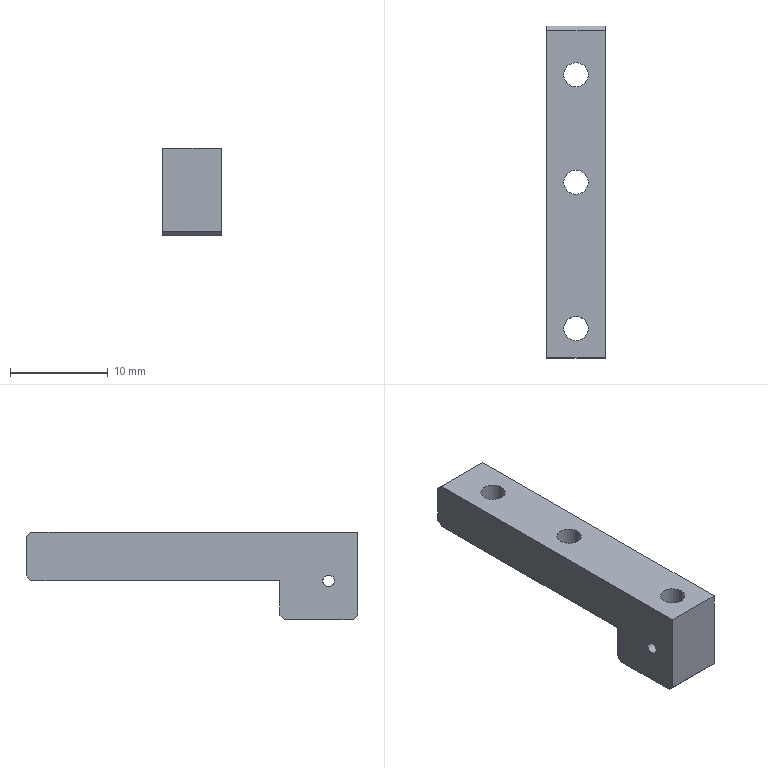Component | SolidWorks | 2018SOLIDWORKS1400000008-1 | 1 solid | 22 faces | box 6 x 34 x 9 mm | volume 1112 mm3 | plane 12 | cylinder 10 | commonest cylinder face diameters 2.5 x6 1.2 x4 | material Brass
build123d program:
from build123d import *

# Parameters (mm, degrees)
SKETCH1_W           = 12
SKETCH1_H           = 4
BOSS_EXTRUDE1_DEPTH = 3
SKETCH10_W          = 34
SKETCH10_H          = 6
BOSS_EXTRUDE2_DEPTH = 5
M3_TAPPED_HOLE1_D   = 2.5
SKETCH9_R           = 0.6
CUT_EXTRUDE7_DEPTH  = 30.479
CHAMFER1_SIZE       = 0.5
SKETCH14_W          = 4
SKETCH14_H          = 6
CUT_EXTRUDE8_DEPTH  = 4
CHAMFER2_SIZE       = 0.5
M3_TAPPED_HOLE2_D   = 2.5


with BuildPart() as part:
    # Sketch1 → Boss-Extrude1 (new, symmetric)
    with BuildSketch(Plane.XY):
        Rectangle(SKETCH1_W, SKETCH1_H)
    extrude(amount=BOSS_EXTRUDE1_DEPTH, both=True)

    # Sketch10 → Boss-Extrude2 (add)
    with BuildSketch(Plane(origin=(0, 2, 0), x_dir=(1, 0, 0), z_dir=(0, 1, 0))):
        with Locations((11, 0)):
            Rectangle(SKETCH10_W, SKETCH10_H)
    extrude(amount=BOSS_EXTRUDE2_DEPTH)

    # M3 Tapped Hole1 (through all)
    with Locations(Plane(origin=(0, 7, 0), x_dir=(1, 0, 0), z_dir=(0, 1, 0))):
        with Locations((12, 0), (23, 0)):
            Hole(M3_TAPPED_HOLE1_D / 2)

    # Sketch9 → Cut-Extrude7 (cut, through all)
    with BuildSketch(Plane.XY.offset(3)):
        with Locations((-3, 2)):
            Circle(SKETCH9_R)
    extrude(amount=-CUT_EXTRUDE7_DEPTH, mode=Mode.SUBTRACT)

    # Chamfer1
    chamfer1_edges = [part.edges().sort_by_distance(p)[0] for p in [
        (28, 7, 0),
        (28, 2, 0),
        (6, -2, 0),
        (-6, -2, 0),
    ]]
    chamfer(chamfer1_edges, length=CHAMFER1_SIZE)

    # Sketch14 → Cut-Extrude8 (cut)
    with BuildSketch(Plane.XZ.offset(2)):
        with Locations((4, 0)):
            Rectangle(SKETCH14_W, SKETCH14_H)
    extrude(amount=-CUT_EXTRUDE8_DEPTH, mode=Mode.SUBTRACT)

    # Chamfer2
    chamfer2_edges = [part.edges().sort_by_distance(p)[0] for p in [
        (2, -2, 0),
    ]]
    chamfer(chamfer2_edges, length=CHAMFER2_SIZE)

    # M3 Tapped Hole2 (through all)
    with Locations(Plane(origin=(0, 7, 0), x_dir=(1, 0, 0), z_dir=(0, 1, 0))):
        with Locations((-3, 0)):
            Hole(M3_TAPPED_HOLE2_D / 2)


solid = part.part

# Placed as in the assembly
solid = solid.moved(Location((84.712, -105.5, 215), (90, 90, 0)))
STEP:
#1=COLOUR_RGB('',0.7922,0.8196,0.9333);
#2=FILL_AREA_STYLE_COLOUR('',#1);
#3=FILL_AREA_STYLE('',(#2));
#4=SURFACE_STYLE_FILL_AREA(#3);
#5=SURFACE_SIDE_STYLE('',(#4));
#6=SURFACE_STYLE_USAGE(.BOTH.,#5);
#7=PRESENTATION_STYLE_ASSIGNMENT((#6));
#8=CARTESIAN_POINT('',(3.286,-4.272,8.386));
#9=VERTEX_POINT('',#8);
#10=CARTESIAN_POINT('',(3.384,-4.272,8.386));
#11=VERTEX_POINT('',#10);
#12=CARTESIAN_POINT('',(3.335,-4.272,8.386));
#13=DIRECTION('',(-0.,0.,1.));
#14=DIRECTION('',(1.,0.,0.));
#15=AXIS2_PLACEMENT_3D('',#12,#13,#14);
#16=CIRCLE('',#15,0.04921);
#17=EDGE_CURVE('',#9,#11,#16,.T.);
#18=ORIENTED_EDGE('',*,*,#17,.F.);
#19=CARTESIAN_POINT('',(3.286,-4.272,8.52));
#20=VERTEX_POINT('',#19);
#21=CARTESIAN_POINT('',(3.286,-4.272,8.74));
#22=DIRECTION('',(-0.,0.,1.));
#23=VECTOR('',#22,39.37);
#24=LINE('',#21,#23);
#25=EDGE_CURVE('',#9,#20,#24,.T.);
#26=ORIENTED_EDGE('',*,*,#25,.T.);
#27=CARTESIAN_POINT('',(3.292,-4.295,8.543));
#28=VERTEX_POINT('',#27);
#29=CARTESIAN_POINT('',(3.292,-4.295,8.543));
#30=CARTESIAN_POINT('',(3.292,-4.295,8.54));
#31=CARTESIAN_POINT('',(3.292,-4.295,8.537));
#32=CARTESIAN_POINT('',(3.29,-4.292,8.531));
#33=CARTESIAN_POINT('',(3.29,-4.291,8.529));
#34=CARTESIAN_POINT('',(3.288,-4.286,8.524));
#35=CARTESIAN_POINT('',(3.287,-4.284,8.523));
#36=CARTESIAN_POINT('',(3.286,-4.278,8.52));
#37=CARTESIAN_POINT('',(3.286,-4.275,8.52));
#38=CARTESIAN_POINT('',(3.286,-4.272,8.52));
#39=B_SPLINE_CURVE_WITH_KNOTS('',3,(#29,#30,#31,#32,#33,#34,#35,#36,#37,#38),.UNSPECIFIED.,.F.,.F.,(4,2,2,2,4),(0.001906,0.002143,0.002381,0.002619,0.002857),.UNSPECIFIED.);
#40=EDGE_CURVE('',#28,#20,#39,.T.);
#41=ORIENTED_EDGE('',*,*,#40,.F.);
#42=CARTESIAN_POINT('',(3.286,-4.272,8.567));
#43=VERTEX_POINT('',#42);
#44=CARTESIAN_POINT('',(3.286,-4.272,8.567));
#45=CARTESIAN_POINT('',(3.286,-4.275,8.567));
#46=CARTESIAN_POINT('',(3.286,-4.278,8.566));
#47=CARTESIAN_POINT('',(3.287,-4.284,8.564));
#48=CARTESIAN_POINT('',(3.288,-4.286,8.562));
#49=CARTESIAN_POINT('',(3.29,-4.291,8.558));
#50=CARTESIAN_POINT('',(3.29,-4.292,8.555));
#51=CARTESIAN_POINT('',(3.292,-4.295,8.55));
#52=CARTESIAN_POINT('',(3.292,-4.295,8.546));
#53=CARTESIAN_POINT('',(3.292,-4.295,8.543));
#54=B_SPLINE_CURVE_WITH_KNOTS('',3,(#44,#45,#46,#47,#48,#49,#50,#51,#52,#53),.UNSPECIFIED.,.F.,.F.,(4,2,2,2,4),(0.0009531,0.001191,0.001429,0.001667,0.001906),.UNSPECIFIED.);
#55=EDGE_CURVE('',#43,#28,#54,.T.);
#56=ORIENTED_EDGE('',*,*,#55,.F.);
#57=CARTESIAN_POINT('',(3.286,-4.272,8.74));
#58=VERTEX_POINT('',#57);
#59=CARTESIAN_POINT('',(3.286,-4.272,8.74));
#60=DIRECTION('',(-0.,0.,1.));
#61=VECTOR('',#60,39.37);
#62=LINE('',#59,#61);
#63=EDGE_CURVE('',#43,#58,#62,.T.);
#64=ORIENTED_EDGE('',*,*,#63,.T.);
#65=CARTESIAN_POINT('',(3.384,-4.272,8.74));
#66=VERTEX_POINT('',#65);
#67=CARTESIAN_POINT('',(3.335,-4.272,8.74));
#68=DIRECTION('',(-0.,0.,1.));
#69=DIRECTION('',(1.,0.,0.));
#70=AXIS2_PLACEMENT_3D('',#67,#68,#69);
#71=CIRCLE('',#70,0.04921);
#72=EDGE_CURVE('',#58,#66,#71,.T.);
#73=ORIENTED_EDGE('',*,*,#72,.T.);
#74=CARTESIAN_POINT('',(3.384,-4.272,8.567));
#75=VERTEX_POINT('',#74);
#76=CARTESIAN_POINT('',(3.384,-4.272,8.74));
#77=DIRECTION('',(-0.,0.,1.));
#78=VECTOR('',#77,39.37);
#79=LINE('',#76,#78);
#80=EDGE_CURVE('',#75,#66,#79,.T.);
#81=ORIENTED_EDGE('',*,*,#80,.F.);
#82=CARTESIAN_POINT('',(3.378,-4.295,8.543));
#83=VERTEX_POINT('',#82);
#84=CARTESIAN_POINT('',(3.378,-4.295,8.543));
#85=CARTESIAN_POINT('',(3.378,-4.295,8.546));
#86=CARTESIAN_POINT('',(3.379,-4.295,8.55));
#87=CARTESIAN_POINT('',(3.38,-4.292,8.555));
#88=CARTESIAN_POINT('',(3.381,-4.291,8.558));
#89=CARTESIAN_POINT('',(3.382,-4.286,8.562));
#90=CARTESIAN_POINT('',(3.383,-4.284,8.564));
#91=CARTESIAN_POINT('',(3.384,-4.278,8.566));
#92=CARTESIAN_POINT('',(3.384,-4.275,8.567));
#93=CARTESIAN_POINT('',(3.384,-4.272,8.567));
#94=B_SPLINE_CURVE_WITH_KNOTS('',3,(#84,#85,#86,#87,#88,#89,#90,#91,#92,#93),.UNSPECIFIED.,.F.,.F.,(4,2,2,2,4),(0.001906,0.002143,0.002381,0.002619,0.002857),.UNSPECIFIED.);
#95=EDGE_CURVE('',#83,#75,#94,.T.);
#96=ORIENTED_EDGE('',*,*,#95,.F.);
#97=CARTESIAN_POINT('',(3.384,-4.272,8.52));
#98=VERTEX_POINT('',#97);
#99=CARTESIAN_POINT('',(3.384,-4.272,8.52));
#100=CARTESIAN_POINT('',(3.384,-4.275,8.52));
#101=CARTESIAN_POINT('',(3.384,-4.278,8.52));
#102=CARTESIAN_POINT('',(3.383,-4.284,8.523));
#103=CARTESIAN_POINT('',(3.382,-4.286,8.524));
#104=CARTESIAN_POINT('',(3.381,-4.291,8.529));
#105=CARTESIAN_POINT('',(3.38,-4.292,8.531));
#106=CARTESIAN_POINT('',(3.379,-4.295,8.537));
#107=CARTESIAN_POINT('',(3.378,-4.295,8.54));
#108=CARTESIAN_POINT('',(3.378,-4.295,8.543));
#109=B_SPLINE_CURVE_WITH_KNOTS('',3,(#99,#100,#101,#102,#103,#104,#105,#106,#107,#108),.UNSPECIFIED.,.F.,.F.,(4,2,2,2,4),(0.0009531,0.001191,0.001429,0.001667,0.001906),.UNSPECIFIED.);
#110=EDGE_CURVE('',#98,#83,#109,.T.);
#111=ORIENTED_EDGE('',*,*,#110,.F.);
#112=CARTESIAN_POINT('',(3.384,-4.272,8.74));
#113=DIRECTION('',(-0.,0.,1.));
#114=VECTOR('',#113,39.37);
#115=LINE('',#112,#114);
#116=EDGE_CURVE('',#11,#98,#115,.T.);
#117=ORIENTED_EDGE('',*,*,#116,.F.);
#118=EDGE_LOOP('',(#18,#26,#41,#56,#64,#73,#81,#96,#111,#117));
#119=FACE_OUTER_BOUND('',#118,.T.);
#120=CARTESIAN_POINT('',(3.335,-4.272,8.74));
#121=DIRECTION('',(-0.,0.,1.));
#122=DIRECTION('',(1.,0.,0.));
#123=AXIS2_PLACEMENT_3D('',#120,#121,#122);
#124=CYLINDRICAL_SURFACE('',#123,0.04921);
#125=ADVANCED_FACE('',(#119),#124,.F.);
#126=CARTESIAN_POINT('',(3.378,-4.248,8.543));
#127=VERTEX_POINT('',#126);
#128=CARTESIAN_POINT('',(3.378,-4.248,8.543));
#129=CARTESIAN_POINT('',(3.378,-4.248,8.537));
#130=CARTESIAN_POINT('',(3.38,-4.251,8.531));
#131=CARTESIAN_POINT('',(3.382,-4.257,8.524));
#132=CARTESIAN_POINT('',(3.383,-4.26,8.523));
#133=CARTESIAN_POINT('',(3.384,-4.265,8.52));
#134=CARTESIAN_POINT('',(3.384,-4.269,8.52));
#135=CARTESIAN_POINT('',(3.384,-4.272,8.52));
#136=B_SPLINE_CURVE_WITH_KNOTS('',3,(#128,#129,#130,#131,#132,#133,#134,#135),.UNSPECIFIED.,.F.,.F.,(4,2,2,4),(0.,0.0004766,0.0007149,0.0009531),.UNSPECIFIED.);
#137=EDGE_CURVE('',#127,#98,#136,.T.);
#138=ORIENTED_EDGE('',*,*,#137,.T.);
#139=ORIENTED_EDGE('',*,*,#110,.T.);
#140=CARTESIAN_POINT('',(3.453,-4.295,8.543));
#141=VERTEX_POINT('',#140);
#142=CARTESIAN_POINT('',(3.217,-4.295,8.543));
#143=DIRECTION('',(1.,-0.,0.));
#144=VECTOR('',#143,39.37);
#145=LINE('',#142,#144);
#146=EDGE_CURVE('',#83,#141,#145,.T.);
#147=ORIENTED_EDGE('',*,*,#146,.T.);
#148=CARTESIAN_POINT('',(3.453,-4.248,8.543));
#149=VERTEX_POINT('',#148);
#150=CARTESIAN_POINT('',(3.453,-4.272,8.543));
#151=DIRECTION('',(1.,-0.,0.));
#152=DIRECTION('',(0.,1.,0.));
#153=AXIS2_PLACEMENT_3D('',#150,#151,#152);
#154=CIRCLE('',#153,0.02362);
#155=EDGE_CURVE('',#141,#149,#154,.T.);
#156=ORIENTED_EDGE('',*,*,#155,.T.);
#157=CARTESIAN_POINT('',(3.217,-4.248,8.543));
#158=DIRECTION('',(1.,-0.,0.));
#159=VECTOR('',#158,39.37);
#160=LINE('',#157,#159);
#161=EDGE_CURVE('',#127,#149,#160,.T.);
#162=ORIENTED_EDGE('',*,*,#161,.F.);
#163=EDGE_LOOP('',(#138,#139,#147,#156,#162));
#164=FACE_OUTER_BOUND('',#163,.T.);
#165=CARTESIAN_POINT('',(3.217,-4.272,8.543));
#166=DIRECTION('',(1.,-0.,0.));
#167=DIRECTION('',(0.,1.,0.));
#168=AXIS2_PLACEMENT_3D('',#165,#166,#167);
#169=CYLINDRICAL_SURFACE('',#168,0.02362);
#170=ADVANCED_FACE('',(#164),#169,.F.);
#171=CARTESIAN_POINT('',(3.286,-3.681,8.543));
#172=VERTEX_POINT('',#171);
#173=CARTESIAN_POINT('',(3.384,-3.681,8.543));
#174=VERTEX_POINT('',#173);
#175=CARTESIAN_POINT('',(3.335,-3.681,8.543));
#176=DIRECTION('',(-0.,0.,1.));
#177=DIRECTION('',(1.,0.,0.));
#178=AXIS2_PLACEMENT_3D('',#175,#176,#177);
#179=CIRCLE('',#178,0.04921);
#180=EDGE_CURVE('',#172,#174,#179,.T.);
#181=ORIENTED_EDGE('',*,*,#180,.F.);
#182=CARTESIAN_POINT('',(3.286,-3.681,8.74));
#183=VERTEX_POINT('',#182);
#184=CARTESIAN_POINT('',(3.286,-3.681,8.74));
#185=DIRECTION('',(-0.,0.,1.));
#186=VECTOR('',#185,39.37);
#187=LINE('',#184,#186);
#188=EDGE_CURVE('',#172,#183,#187,.T.);
#189=ORIENTED_EDGE('',*,*,#188,.T.);
#190=CARTESIAN_POINT('',(3.384,-3.681,8.74));
#191=VERTEX_POINT('',#190);
#192=CARTESIAN_POINT('',(3.335,-3.681,8.74));
#193=DIRECTION('',(-0.,0.,1.));
#194=DIRECTION('',(1.,0.,0.));
#195=AXIS2_PLACEMENT_3D('',#192,#193,#194);
#196=CIRCLE('',#195,0.04921);
#197=EDGE_CURVE('',#183,#191,#196,.T.);
#198=ORIENTED_EDGE('',*,*,#197,.T.);
#199=CARTESIAN_POINT('',(3.384,-3.681,8.74));
#200=DIRECTION('',(-0.,0.,1.));
#201=VECTOR('',#200,39.37);
#202=LINE('',#199,#201);
#203=EDGE_CURVE('',#174,#191,#202,.T.);
#204=ORIENTED_EDGE('',*,*,#203,.F.);
#205=EDGE_LOOP('',(#181,#189,#198,#204));
#206=FACE_OUTER_BOUND('',#205,.T.);
#207=CARTESIAN_POINT('',(3.335,-3.681,8.74));
#208=DIRECTION('',(-0.,0.,1.));
#209=DIRECTION('',(1.,0.,0.));
#210=AXIS2_PLACEMENT_3D('',#207,#208,#209);
#211=CYLINDRICAL_SURFACE('',#210,0.04921);
#212=ADVANCED_FACE('',(#206),#211,.F.);
#213=CARTESIAN_POINT('',(3.286,-3.248,8.543));
#214=VERTEX_POINT('',#213);
#215=CARTESIAN_POINT('',(3.384,-3.248,8.543));
#216=VERTEX_POINT('',#215);
#217=CARTESIAN_POINT('',(3.335,-3.248,8.543));
#218=DIRECTION('',(-0.,0.,1.));
#219=DIRECTION('',(1.,0.,0.));
#220=AXIS2_PLACEMENT_3D('',#217,#218,#219);
#221=CIRCLE('',#220,0.04921);
#222=EDGE_CURVE('',#214,#216,#221,.T.);
#223=ORIENTED_EDGE('',*,*,#222,.F.);
#224=CARTESIAN_POINT('',(3.286,-3.248,8.74));
#225=VERTEX_POINT('',#224);
#226=CARTESIAN_POINT('',(3.286,-3.248,8.74));
#227=DIRECTION('',(-0.,0.,1.));
#228=VECTOR('',#227,39.37);
#229=LINE('',#226,#228);
#230=EDGE_CURVE('',#214,#225,#229,.T.);
#231=ORIENTED_EDGE('',*,*,#230,.T.);
#232=CARTESIAN_POINT('',(3.384,-3.248,8.74));
#233=VERTEX_POINT('',#232);
#234=CARTESIAN_POINT('',(3.335,-3.248,8.74));
#235=DIRECTION('',(-0.,0.,1.));
#236=DIRECTION('',(1.,0.,0.));
#237=AXIS2_PLACEMENT_3D('',#234,#235,#236);
#238=CIRCLE('',#237,0.04921);
#239=EDGE_CURVE('',#225,#233,#238,.T.);
#240=ORIENTED_EDGE('',*,*,#239,.T.);
#241=CARTESIAN_POINT('',(3.384,-3.248,8.74));
#242=DIRECTION('',(-0.,0.,1.));
#243=VECTOR('',#242,39.37);
#244=LINE('',#241,#243);
#245=EDGE_CURVE('',#216,#233,#244,.T.);
#246=ORIENTED_EDGE('',*,*,#245,.F.);
#247=EDGE_LOOP('',(#223,#231,#240,#246));
#248=FACE_OUTER_BOUND('',#247,.T.);
#249=CARTESIAN_POINT('',(3.335,-3.248,8.74));
#250=DIRECTION('',(-0.,0.,1.));
#251=DIRECTION('',(1.,0.,0.));
#252=AXIS2_PLACEMENT_3D('',#249,#250,#251);
#253=CYLINDRICAL_SURFACE('',#252,0.04921);
#254=ADVANCED_FACE('',(#248),#253,.F.);
#255=CARTESIAN_POINT('',(3.217,-4.295,8.543));
#256=VERTEX_POINT('',#255);
#257=CARTESIAN_POINT('',(3.217,-4.248,8.543));
#258=VERTEX_POINT('',#257);
#259=CARTESIAN_POINT('',(3.217,-4.272,8.543));
#260=DIRECTION('',(1.,-0.,0.));
#261=DIRECTION('',(0.,1.,0.));
#262=AXIS2_PLACEMENT_3D('',#259,#260,#261);
#263=CIRCLE('',#262,0.02362);
#264=EDGE_CURVE('',#256,#258,#263,.T.);
#265=ORIENTED_EDGE('',*,*,#264,.F.);
#266=CARTESIAN_POINT('',(3.217,-4.295,8.543));
#267=DIRECTION('',(1.,-0.,0.));
#268=VECTOR('',#267,39.37);
#269=LINE('',#266,#268);
#270=EDGE_CURVE('',#256,#28,#269,.T.);
#271=ORIENTED_EDGE('',*,*,#270,.T.);
#272=ORIENTED_EDGE('',*,*,#40,.T.);
#273=CARTESIAN_POINT('',(3.292,-4.248,8.543));
#274=VERTEX_POINT('',#273);
#275=CARTESIAN_POINT('',(3.286,-4.272,8.52));
#276=CARTESIAN_POINT('',(3.286,-4.269,8.52));
#277=CARTESIAN_POINT('',(3.286,-4.265,8.52));
#278=CARTESIAN_POINT('',(3.287,-4.26,8.523));
#279=CARTESIAN_POINT('',(3.288,-4.257,8.524));
#280=CARTESIAN_POINT('',(3.29,-4.251,8.531));
#281=CARTESIAN_POINT('',(3.292,-4.248,8.537));
#282=CARTESIAN_POINT('',(3.292,-4.248,8.543));
#283=B_SPLINE_CURVE_WITH_KNOTS('',3,(#275,#276,#277,#278,#279,#280,#281,#282),.UNSPECIFIED.,.F.,.F.,(4,2,2,4),(0.002857,0.003095,0.003333,0.003808),.UNSPECIFIED.);
#284=EDGE_CURVE('',#20,#274,#283,.T.);
#285=ORIENTED_EDGE('',*,*,#284,.T.);
#286=CARTESIAN_POINT('',(3.217,-4.248,8.543));
#287=DIRECTION('',(1.,-0.,0.));
#288=VECTOR('',#287,39.37);
#289=LINE('',#286,#288);
#290=EDGE_CURVE('',#258,#274,#289,.T.);
#291=ORIENTED_EDGE('',*,*,#290,.F.);
#292=EDGE_LOOP('',(#265,#271,#272,#285,#291));
#293=FACE_OUTER_BOUND('',#292,.T.);
#294=CARTESIAN_POINT('',(3.217,-4.272,8.543));
#295=DIRECTION('',(1.,-0.,0.));
#296=DIRECTION('',(0.,1.,0.));
#297=AXIS2_PLACEMENT_3D('',#294,#295,#296);
#298=CYLINDRICAL_SURFACE('',#297,0.02362);
#299=ADVANCED_FACE('',(#293),#298,.F.);
#300=ORIENTED_EDGE('',*,*,#270,.F.);
#301=CARTESIAN_POINT('',(3.217,-4.272,8.543));
#302=DIRECTION('',(1.,-0.,0.));
#303=DIRECTION('',(0.,1.,0.));
#304=AXIS2_PLACEMENT_3D('',#301,#302,#303);
#305=CIRCLE('',#304,0.02362);
#306=EDGE_CURVE('',#258,#256,#305,.T.);
#307=ORIENTED_EDGE('',*,*,#306,.F.);
#308=ORIENTED_EDGE('',*,*,#290,.T.);
#309=CARTESIAN_POINT('',(3.292,-4.248,8.543));
#310=CARTESIAN_POINT('',(3.292,-4.248,8.55));
#311=CARTESIAN_POINT('',(3.29,-4.251,8.556));
#312=CARTESIAN_POINT('',(3.288,-4.257,8.562));
#313=CARTESIAN_POINT('',(3.287,-4.26,8.564));
#314=CARTESIAN_POINT('',(3.286,-4.265,8.566));
#315=CARTESIAN_POINT('',(3.286,-4.269,8.567));
#316=CARTESIAN_POINT('',(3.286,-4.272,8.567));
#317=B_SPLINE_CURVE_WITH_KNOTS('',3,(#309,#310,#311,#312,#313,#314,#315,#316),.UNSPECIFIED.,.F.,.F.,(4,2,2,4),(0.,0.0004766,0.0007149,0.0009531),.UNSPECIFIED.);
#318=EDGE_CURVE('',#274,#43,#317,.T.);
#319=ORIENTED_EDGE('',*,*,#318,.T.);
#320=ORIENTED_EDGE('',*,*,#55,.T.);
#321=EDGE_LOOP('',(#300,#307,#308,#319,#320));
#322=FACE_OUTER_BOUND('',#321,.T.);
#323=CARTESIAN_POINT('',(3.217,-4.272,8.543));
#324=DIRECTION('',(1.,-0.,0.));
#325=DIRECTION('',(0.,1.,0.));
#326=AXIS2_PLACEMENT_3D('',#323,#324,#325);
#327=CYLINDRICAL_SURFACE('',#326,0.02362);
#328=ADVANCED_FACE('',(#322),#327,.F.);
#329=CARTESIAN_POINT('',(3.217,-4.39,8.74));
#330=VERTEX_POINT('',#329);
#331=CARTESIAN_POINT('',(3.217,-4.39,8.406));
#332=VERTEX_POINT('',#331);
#333=CARTESIAN_POINT('',(3.217,-4.39,8.543));
#334=DIRECTION('',(0.,-0.,-1.));
#335=VECTOR('',#334,39.37);
#336=LINE('',#333,#335);
#337=EDGE_CURVE('',#330,#332,#336,.T.);
#338=ORIENTED_EDGE('',*,*,#337,.T.);
#339=CARTESIAN_POINT('',(3.453,-4.39,8.406));
#340=VERTEX_POINT('',#339);
#341=CARTESIAN_POINT('',(3.453,-4.39,8.406));
#342=DIRECTION('',(1.,-0.,0.));
#343=VECTOR('',#342,39.37);
#344=LINE('',#341,#343);
#345=EDGE_CURVE('',#332,#340,#344,.T.);
#346=ORIENTED_EDGE('',*,*,#345,.T.);
#347=CARTESIAN_POINT('',(3.453,-4.39,8.74));
#348=VERTEX_POINT('',#347);
#349=CARTESIAN_POINT('',(3.453,-4.39,8.543));
#350=DIRECTION('',(0.,-0.,-1.));
#351=VECTOR('',#350,39.37);
#352=LINE('',#349,#351);
#353=EDGE_CURVE('',#348,#340,#352,.T.);
#354=ORIENTED_EDGE('',*,*,#353,.F.);
#355=CARTESIAN_POINT('',(3.217,-4.39,8.74));
#356=DIRECTION('',(1.,0.,0.));
#357=VECTOR('',#356,39.37);
#358=LINE('',#355,#357);
#359=EDGE_CURVE('',#330,#348,#358,.T.);
#360=ORIENTED_EDGE('',*,*,#359,.F.);
#361=EDGE_LOOP('',(#338,#346,#354,#360));
#362=FACE_OUTER_BOUND('',#361,.T.);
#363=CARTESIAN_POINT('',(3.453,-4.39,8.543));
#364=DIRECTION('',(-0.,1.,-0.));
#365=DIRECTION('',(-0.,0.,1.));
#366=AXIS2_PLACEMENT_3D('',#363,#364,#365);
#367=PLANE('',#366);
#368=ADVANCED_FACE('',(#362),#367,.F.);
#369=CARTESIAN_POINT('',(3.335,-4.272,8.386));
#370=DIRECTION('',(-0.,0.,1.));
#371=DIRECTION('',(1.,0.,0.));
#372=AXIS2_PLACEMENT_3D('',#369,#370,#371);
#373=CIRCLE('',#372,0.04921);
#374=EDGE_CURVE('',#11,#9,#373,.T.);
#375=ORIENTED_EDGE('',*,*,#374,.T.);
#376=ORIENTED_EDGE('',*,*,#17,.T.);
#377=EDGE_LOOP('',(#375,#376));
#378=FACE_BOUND('',#377,.T.);
#379=CARTESIAN_POINT('',(3.217,-4.37,8.386));
#380=VERTEX_POINT('',#379);
#381=CARTESIAN_POINT('',(3.217,-4.094,8.386));
#382=VERTEX_POINT('',#381);
#383=CARTESIAN_POINT('',(3.217,-4.39,8.386));
#384=DIRECTION('',(-0.,1.,-0.));
#385=VECTOR('',#384,39.37);
#386=LINE('',#383,#385);
#387=EDGE_CURVE('',#380,#382,#386,.T.);
#388=ORIENTED_EDGE('',*,*,#387,.T.);
#389=CARTESIAN_POINT('',(3.453,-4.094,8.386));
#390=VERTEX_POINT('',#389);
#391=CARTESIAN_POINT('',(3.453,-4.094,8.386));
#392=DIRECTION('',(1.,-0.,0.));
#393=VECTOR('',#392,39.37);
#394=LINE('',#391,#393);
#395=EDGE_CURVE('',#382,#390,#394,.T.);
#396=ORIENTED_EDGE('',*,*,#395,.T.);
#397=CARTESIAN_POINT('',(3.453,-4.37,8.386));
#398=VERTEX_POINT('',#397);
#399=CARTESIAN_POINT('',(3.453,-4.39,8.386));
#400=DIRECTION('',(-0.,1.,-0.));
#401=VECTOR('',#400,39.37);
#402=LINE('',#399,#401);
#403=EDGE_CURVE('',#398,#390,#402,.T.);
#404=ORIENTED_EDGE('',*,*,#403,.F.);
#405=CARTESIAN_POINT('',(3.453,-4.37,8.386));
#406=DIRECTION('',(-1.,0.,-0.));
#407=VECTOR('',#406,39.37);
#408=LINE('',#405,#407);
#409=EDGE_CURVE('',#398,#380,#408,.T.);
#410=ORIENTED_EDGE('',*,*,#409,.T.);
#411=EDGE_LOOP('',(#388,#396,#404,#410));
#412=FACE_OUTER_BOUND('',#411,.T.);
#413=CARTESIAN_POINT('',(3.453,-4.39,8.386));
#414=DIRECTION('',(-0.,0.,1.));
#415=DIRECTION('',(1.,-0.,0.));
#416=AXIS2_PLACEMENT_3D('',#413,#414,#415);
#417=PLANE('',#416);
#418=ADVANCED_FACE('',(#378,#412),#417,.F.);
#419=ORIENTED_EDGE('',*,*,#403,.T.);
#420=CARTESIAN_POINT('',(3.453,-4.075,8.406));
#421=VERTEX_POINT('',#420);
#422=CARTESIAN_POINT('',(3.453,-4.085,8.396));
#423=DIRECTION('',(-0.,0.7071,0.7071));
#424=VECTOR('',#423,39.37);
#425=LINE('',#422,#424);
#426=EDGE_CURVE('',#390,#421,#425,.T.);
#427=ORIENTED_EDGE('',*,*,#426,.T.);
#428=CARTESIAN_POINT('',(3.453,-4.075,8.543));
#429=VERTEX_POINT('',#428);
#430=CARTESIAN_POINT('',(3.453,-4.075,8.827));
#431=DIRECTION('',(0.,-0.,-1.));
#432=VECTOR('',#431,39.37);
#433=LINE('',#430,#432);
#434=EDGE_CURVE('',#429,#421,#433,.T.);
#435=ORIENTED_EDGE('',*,*,#434,.F.);
#436=CARTESIAN_POINT('',(3.453,-3.071,8.543));
#437=VERTEX_POINT('',#436);
#438=CARTESIAN_POINT('',(3.453,-4.39,8.543));
#439=DIRECTION('',(-0.,1.,-0.));
#440=VECTOR('',#439,39.37);
#441=LINE('',#438,#440);
#442=EDGE_CURVE('',#429,#437,#441,.T.);
#443=ORIENTED_EDGE('',*,*,#442,.T.);
#444=CARTESIAN_POINT('',(3.453,-3.051,8.563));
#445=VERTEX_POINT('',#444);
#446=CARTESIAN_POINT('',(3.453,-3.652,7.963));
#447=DIRECTION('',(-0.,0.7071,0.7071));
#448=VECTOR('',#447,39.37);
#449=LINE('',#446,#448);
#450=EDGE_CURVE('',#437,#445,#449,.T.);
#451=ORIENTED_EDGE('',*,*,#450,.T.);
#452=CARTESIAN_POINT('',(3.453,-3.051,8.72));
#453=VERTEX_POINT('',#452);
#454=CARTESIAN_POINT('',(3.453,-3.051,8.74));
#455=DIRECTION('',(0.,-0.,-1.));
#456=VECTOR('',#455,39.37);
#457=LINE('',#454,#456);
#458=EDGE_CURVE('',#453,#445,#457,.T.);
#459=ORIENTED_EDGE('',*,*,#458,.F.);
#460=CARTESIAN_POINT('',(3.453,-3.071,8.74));
#461=VERTEX_POINT('',#460);
#462=CARTESIAN_POINT('',(3.453,-3.474,9.144));
#463=DIRECTION('',(-0.,-0.7071,0.7071));
#464=VECTOR('',#463,39.37);
#465=LINE('',#462,#464);
#466=EDGE_CURVE('',#453,#461,#465,.T.);
#467=ORIENTED_EDGE('',*,*,#466,.T.);
#468=CARTESIAN_POINT('',(3.453,-4.39,8.74));
#469=DIRECTION('',(-0.,1.,-0.));
#470=VECTOR('',#469,39.37);
#471=LINE('',#468,#470);
#472=EDGE_CURVE('',#348,#461,#471,.T.);
#473=ORIENTED_EDGE('',*,*,#472,.F.);
#474=ORIENTED_EDGE('',*,*,#353,.T.);
#475=CARTESIAN_POINT('',(3.453,-4.301,8.317));
#476=DIRECTION('',(0.,0.7071,-0.7071));
#477=VECTOR('',#476,39.37);
#478=LINE('',#475,#477);
#479=EDGE_CURVE('',#340,#398,#478,.T.);
#480=ORIENTED_EDGE('',*,*,#479,.T.);
#481=EDGE_LOOP('',(#419,#427,#435,#443,#451,#459,#467,#473,#474,#480));
#482=FACE_OUTER_BOUND('',#481,.T.);
#483=CARTESIAN_POINT('',(3.453,-4.272,8.543));
#484=DIRECTION('',(1.,-0.,0.));
#485=DIRECTION('',(0.,1.,0.));
#486=AXIS2_PLACEMENT_3D('',#483,#484,#485);
#487=CIRCLE('',#486,0.02362);
#488=EDGE_CURVE('',#149,#141,#487,.T.);
#489=ORIENTED_EDGE('',*,*,#488,.F.);
#490=ORIENTED_EDGE('',*,*,#155,.F.);
#491=EDGE_LOOP('',(#489,#490));
#492=FACE_BOUND('',#491,.T.);
#493=CARTESIAN_POINT('',(3.453,-4.154,8.465));
#494=DIRECTION('',(1.,0.,0.));
#495=DIRECTION('',(-0.,1.,-0.));
#496=AXIS2_PLACEMENT_3D('',#493,#494,#495);
#497=PLANE('',#496);
#498=ADVANCED_FACE('',(#482,#492),#497,.T.);
#499=ORIENTED_EDGE('',*,*,#306,.T.);
#500=ORIENTED_EDGE('',*,*,#264,.T.);
#501=EDGE_LOOP('',(#499,#500));
#502=FACE_BOUND('',#501,.T.);
#503=CARTESIAN_POINT('',(3.217,-4.075,8.543));
#504=VERTEX_POINT('',#503);
#505=CARTESIAN_POINT('',(3.217,-4.075,8.406));
#506=VERTEX_POINT('',#505);
#507=CARTESIAN_POINT('',(3.217,-4.075,8.827));
#508=DIRECTION('',(0.,-0.,-1.));
#509=VECTOR('',#508,39.37);
#510=LINE('',#507,#509);
#511=EDGE_CURVE('',#504,#506,#510,.T.);
#512=ORIENTED_EDGE('',*,*,#511,.T.);
#513=CARTESIAN_POINT('',(3.217,-4.075,8.406));
#514=DIRECTION('',(0.,-0.7071,-0.7071));
#515=VECTOR('',#514,39.37);
#516=LINE('',#513,#515);
#517=EDGE_CURVE('',#506,#382,#516,.T.);
#518=ORIENTED_EDGE('',*,*,#517,.T.);
#519=ORIENTED_EDGE('',*,*,#387,.F.);
#520=CARTESIAN_POINT('',(3.217,-4.37,8.386));
#521=DIRECTION('',(-0.,-0.7071,0.7071));
#522=VECTOR('',#521,39.37);
#523=LINE('',#520,#522);
#524=EDGE_CURVE('',#380,#332,#523,.T.);
#525=ORIENTED_EDGE('',*,*,#524,.T.);
#526=ORIENTED_EDGE('',*,*,#337,.F.);
#527=CARTESIAN_POINT('',(3.217,-3.071,8.74));
#528=VERTEX_POINT('',#527);
#529=CARTESIAN_POINT('',(3.217,-4.39,8.74));
#530=DIRECTION('',(0.,-1.,0.));
#531=VECTOR('',#530,39.37);
#532=LINE('',#529,#531);
#533=EDGE_CURVE('',#528,#330,#532,.T.);
#534=ORIENTED_EDGE('',*,*,#533,.F.);
#535=CARTESIAN_POINT('',(3.217,-3.051,8.72));
#536=VERTEX_POINT('',#535);
#537=CARTESIAN_POINT('',(3.217,-3.071,8.74));
#538=DIRECTION('',(0.,0.7071,-0.7071));
#539=VECTOR('',#538,39.37);
#540=LINE('',#537,#539);
#541=EDGE_CURVE('',#528,#536,#540,.T.);
#542=ORIENTED_EDGE('',*,*,#541,.T.);
#543=CARTESIAN_POINT('',(3.217,-3.051,8.563));
#544=VERTEX_POINT('',#543);
#545=CARTESIAN_POINT('',(3.217,-3.051,8.74));
#546=DIRECTION('',(0.,-0.,-1.));
#547=VECTOR('',#546,39.37);
#548=LINE('',#545,#547);
#549=EDGE_CURVE('',#536,#544,#548,.T.);
#550=ORIENTED_EDGE('',*,*,#549,.T.);
#551=CARTESIAN_POINT('',(3.217,-3.071,8.543));
#552=VERTEX_POINT('',#551);
#553=CARTESIAN_POINT('',(3.217,-3.051,8.563));
#554=DIRECTION('',(0.,-0.7071,-0.7071));
#555=VECTOR('',#554,39.37);
#556=LINE('',#553,#555);
#557=EDGE_CURVE('',#544,#552,#556,.T.);
#558=ORIENTED_EDGE('',*,*,#557,.T.);
#559=CARTESIAN_POINT('',(3.217,-4.39,8.543));
#560=DIRECTION('',(0.,-1.,0.));
#561=VECTOR('',#560,39.37);
#562=LINE('',#559,#561);
#563=EDGE_CURVE('',#552,#504,#562,.T.);
#564=ORIENTED_EDGE('',*,*,#563,.T.);
#565=EDGE_LOOP('',(#512,#518,#519,#525,#526,#534,#542,#550,#558,#564));
#566=FACE_OUTER_BOUND('',#565,.T.);
#567=CARTESIAN_POINT('',(3.217,-4.154,8.465));
#568=DIRECTION('',(1.,0.,0.));
#569=DIRECTION('',(-0.,1.,-0.));
#570=AXIS2_PLACEMENT_3D('',#567,#568,#569);
#571=PLANE('',#570);
#572=ADVANCED_FACE('',(#502,#566),#571,.F.);
#573=CARTESIAN_POINT('',(3.335,-3.681,8.543));
#574=DIRECTION('',(-0.,0.,1.));
#575=DIRECTION('',(1.,0.,0.));
#576=AXIS2_PLACEMENT_3D('',#573,#574,#575);
#577=CIRCLE('',#576,0.04921);
#578=EDGE_CURVE('',#174,#172,#577,.T.);
#579=ORIENTED_EDGE('',*,*,#578,.T.);
#580=ORIENTED_EDGE('',*,*,#180,.T.);
#581=EDGE_LOOP('',(#579,#580));
#582=FACE_BOUND('',#581,.T.);
#583=CARTESIAN_POINT('',(3.335,-3.248,8.543));
#584=DIRECTION('',(-0.,0.,1.));
#585=DIRECTION('',(1.,0.,0.));
#586=AXIS2_PLACEMENT_3D('',#583,#584,#585);
#587=CIRCLE('',#586,0.04921);
#588=EDGE_CURVE('',#216,#214,#587,.T.);
#589=ORIENTED_EDGE('',*,*,#588,.T.);
#590=ORIENTED_EDGE('',*,*,#222,.T.);
#591=EDGE_LOOP('',(#589,#590));
#592=FACE_BOUND('',#591,.T.);
#593=ORIENTED_EDGE('',*,*,#563,.F.);
#594=CARTESIAN_POINT('',(3.335,-3.071,8.543));
#595=DIRECTION('',(1.,-0.,0.));
#596=VECTOR('',#595,39.37);
#597=LINE('',#594,#596);
#598=EDGE_CURVE('',#552,#437,#597,.T.);
#599=ORIENTED_EDGE('',*,*,#598,.T.);
#600=ORIENTED_EDGE('',*,*,#442,.F.);
#601=CARTESIAN_POINT('',(3.217,-4.075,8.543));
#602=DIRECTION('',(-1.,0.,-0.));
#603=VECTOR('',#602,39.37);
#604=LINE('',#601,#603);
#605=EDGE_CURVE('',#429,#504,#604,.T.);
#606=ORIENTED_EDGE('',*,*,#605,.T.);
#607=EDGE_LOOP('',(#593,#599,#600,#606));
#608=FACE_OUTER_BOUND('',#607,.T.);
#609=CARTESIAN_POINT('',(3.335,-4.154,8.543));
#610=DIRECTION('',(-0.,0.,1.));
#611=DIRECTION('',(1.,-0.,0.));
#612=AXIS2_PLACEMENT_3D('',#609,#610,#611);
#613=PLANE('',#612);
#614=ADVANCED_FACE('',(#582,#592,#608),#613,.F.);
#615=ORIENTED_EDGE('',*,*,#549,.F.);
#616=CARTESIAN_POINT('',(3.453,-3.051,8.72));
#617=DIRECTION('',(1.,-0.,0.));
#618=VECTOR('',#617,39.37);
#619=LINE('',#616,#618);
#620=EDGE_CURVE('',#536,#453,#619,.T.);
#621=ORIENTED_EDGE('',*,*,#620,.T.);
#622=ORIENTED_EDGE('',*,*,#458,.T.);
#623=CARTESIAN_POINT('',(3.217,-3.051,8.563));
#624=DIRECTION('',(-1.,0.,-0.));
#625=VECTOR('',#624,39.37);
#626=LINE('',#623,#625);
#627=EDGE_CURVE('',#445,#544,#626,.T.);
#628=ORIENTED_EDGE('',*,*,#627,.T.);
#629=EDGE_LOOP('',(#615,#621,#622,#628));
#630=FACE_OUTER_BOUND('',#629,.T.);
#631=CARTESIAN_POINT('',(3.217,-3.051,8.74));
#632=DIRECTION('',(-0.,-1.,0.));
#633=DIRECTION('',(1.,-0.,0.));
#634=AXIS2_PLACEMENT_3D('',#631,#632,#633);
#635=PLANE('',#634);
#636=ADVANCED_FACE('',(#630),#635,.F.);
#637=CARTESIAN_POINT('',(3.335,-4.272,8.74));
#638=DIRECTION('',(-0.,0.,1.));
#639=DIRECTION('',(1.,0.,0.));
#640=AXIS2_PLACEMENT_3D('',#637,#638,#639);
#641=CIRCLE('',#640,0.04921);
#642=EDGE_CURVE('',#66,#58,#641,.T.);
#643=ORIENTED_EDGE('',*,*,#642,.F.);
#644=ORIENTED_EDGE('',*,*,#72,.F.);
#645=EDGE_LOOP('',(#643,#644));
#646=FACE_BOUND('',#645,.T.);
#647=CARTESIAN_POINT('',(3.335,-3.681,8.74));
#648=DIRECTION('',(-0.,0.,1.));
#649=DIRECTION('',(1.,0.,0.));
#650=AXIS2_PLACEMENT_3D('',#647,#648,#649);
#651=CIRCLE('',#650,0.04921);
#652=EDGE_CURVE('',#191,#183,#651,.T.);
#653=ORIENTED_EDGE('',*,*,#652,.F.);
#654=ORIENTED_EDGE('',*,*,#197,.F.);
#655=EDGE_LOOP('',(#653,#654));
#656=FACE_BOUND('',#655,.T.);
#657=CARTESIAN_POINT('',(3.335,-3.248,8.74));
#658=DIRECTION('',(-0.,0.,1.));
#659=DIRECTION('',(1.,0.,0.));
#660=AXIS2_PLACEMENT_3D('',#657,#658,#659);
#661=CIRCLE('',#660,0.04921);
#662=EDGE_CURVE('',#233,#225,#661,.T.);
#663=ORIENTED_EDGE('',*,*,#662,.F.);
#664=ORIENTED_EDGE('',*,*,#239,.F.);
#665=EDGE_LOOP('',(#663,#664));
#666=FACE_BOUND('',#665,.T.);
#667=ORIENTED_EDGE('',*,*,#472,.T.);
#668=CARTESIAN_POINT('',(3.217,-3.071,8.74));
#669=DIRECTION('',(-1.,0.,-0.));
#670=VECTOR('',#669,39.37);
#671=LINE('',#668,#670);
#672=EDGE_CURVE('',#461,#528,#671,.T.);
#673=ORIENTED_EDGE('',*,*,#672,.T.);
#674=ORIENTED_EDGE('',*,*,#533,.T.);
#675=ORIENTED_EDGE('',*,*,#359,.T.);
#676=EDGE_LOOP('',(#667,#673,#674,#675));
#677=FACE_OUTER_BOUND('',#676,.T.);
#678=CARTESIAN_POINT('',(3.335,-4.154,8.74));
#679=DIRECTION('',(-0.,0.,1.));
#680=DIRECTION('',(1.,-0.,0.));
#681=AXIS2_PLACEMENT_3D('',#678,#679,#680);
#682=PLANE('',#681);
#683=ADVANCED_FACE('',(#646,#656,#666,#677),#682,.T.);
#684=ORIENTED_EDGE('',*,*,#230,.F.);
#685=ORIENTED_EDGE('',*,*,#588,.F.);
#686=ORIENTED_EDGE('',*,*,#245,.T.);
#687=ORIENTED_EDGE('',*,*,#662,.T.);
#688=EDGE_LOOP('',(#684,#685,#686,#687));
#689=FACE_OUTER_BOUND('',#688,.T.);
#690=CARTESIAN_POINT('',(3.335,-3.248,8.74));
#691=DIRECTION('',(-0.,0.,1.));
#692=DIRECTION('',(1.,0.,0.));
#693=AXIS2_PLACEMENT_3D('',#690,#691,#692);
#694=CYLINDRICAL_SURFACE('',#693,0.04921);
#695=ADVANCED_FACE('',(#689),#694,.F.);
#696=ORIENTED_EDGE('',*,*,#188,.F.);
#697=ORIENTED_EDGE('',*,*,#578,.F.);
#698=ORIENTED_EDGE('',*,*,#203,.T.);
#699=ORIENTED_EDGE('',*,*,#652,.T.);
#700=EDGE_LOOP('',(#696,#697,#698,#699));
#701=FACE_OUTER_BOUND('',#700,.T.);
#702=CARTESIAN_POINT('',(3.335,-3.681,8.74));
#703=DIRECTION('',(-0.,0.,1.));
#704=DIRECTION('',(1.,0.,0.));
#705=AXIS2_PLACEMENT_3D('',#702,#703,#704);
#706=CYLINDRICAL_SURFACE('',#705,0.04921);
#707=ADVANCED_FACE('',(#701),#706,.F.);
#708=ORIENTED_EDGE('',*,*,#146,.F.);
#709=ORIENTED_EDGE('',*,*,#95,.T.);
#710=CARTESIAN_POINT('',(3.384,-4.272,8.567));
#711=CARTESIAN_POINT('',(3.384,-4.269,8.567));
#712=CARTESIAN_POINT('',(3.384,-4.265,8.566));
#713=CARTESIAN_POINT('',(3.383,-4.26,8.564));
#714=CARTESIAN_POINT('',(3.382,-4.257,8.562));
#715=CARTESIAN_POINT('',(3.38,-4.251,8.556));
#716=CARTESIAN_POINT('',(3.378,-4.248,8.55));
#717=CARTESIAN_POINT('',(3.378,-4.248,8.543));
#718=B_SPLINE_CURVE_WITH_KNOTS('',3,(#710,#711,#712,#713,#714,#715,#716,#717),.UNSPECIFIED.,.F.,.F.,(4,2,2,4),(0.002857,0.003095,0.003333,0.003808),.UNSPECIFIED.);
#719=EDGE_CURVE('',#75,#127,#718,.T.);
#720=ORIENTED_EDGE('',*,*,#719,.T.);
#721=ORIENTED_EDGE('',*,*,#161,.T.);
#722=ORIENTED_EDGE('',*,*,#488,.T.);
#723=EDGE_LOOP('',(#708,#709,#720,#721,#722));
#724=FACE_OUTER_BOUND('',#723,.T.);
#725=CARTESIAN_POINT('',(3.217,-4.272,8.543));
#726=DIRECTION('',(1.,-0.,0.));
#727=DIRECTION('',(0.,1.,0.));
#728=AXIS2_PLACEMENT_3D('',#725,#726,#727);
#729=CYLINDRICAL_SURFACE('',#728,0.02362);
#730=ADVANCED_FACE('',(#724),#729,.F.);
#731=ORIENTED_EDGE('',*,*,#466,.F.);
#732=ORIENTED_EDGE('',*,*,#620,.F.);
#733=ORIENTED_EDGE('',*,*,#541,.F.);
#734=ORIENTED_EDGE('',*,*,#672,.F.);
#735=EDGE_LOOP('',(#731,#732,#733,#734));
#736=FACE_OUTER_BOUND('',#735,.T.);
#737=CARTESIAN_POINT('',(3.335,-3.071,8.74));
#738=DIRECTION('',(-0.,0.7071,0.7071));
#739=DIRECTION('',(1.,-0.,0.));
#740=AXIS2_PLACEMENT_3D('',#737,#738,#739);
#741=PLANE('',#740);
#742=ADVANCED_FACE('',(#736),#741,.T.);
#743=ORIENTED_EDGE('',*,*,#450,.F.);
#744=ORIENTED_EDGE('',*,*,#598,.F.);
#745=ORIENTED_EDGE('',*,*,#557,.F.);
#746=ORIENTED_EDGE('',*,*,#627,.F.);
#747=EDGE_LOOP('',(#743,#744,#745,#746));
#748=FACE_OUTER_BOUND('',#747,.T.);
#749=CARTESIAN_POINT('',(3.217,-3.051,8.563));
#750=DIRECTION('',(-0.,-0.7071,0.7071));
#751=DIRECTION('',(-1.,0.,-0.));
#752=AXIS2_PLACEMENT_3D('',#749,#750,#751);
#753=PLANE('',#752);
#754=ADVANCED_FACE('',(#748),#753,.F.);
#755=ORIENTED_EDGE('',*,*,#479,.F.);
#756=ORIENTED_EDGE('',*,*,#345,.F.);
#757=ORIENTED_EDGE('',*,*,#524,.F.);
#758=ORIENTED_EDGE('',*,*,#409,.F.);
#759=EDGE_LOOP('',(#755,#756,#757,#758));
#760=FACE_OUTER_BOUND('',#759,.T.);
#761=CARTESIAN_POINT('',(3.453,-4.37,8.386));
#762=DIRECTION('',(-0.,0.7071,0.7071));
#763=DIRECTION('',(-1.,0.,-0.));
#764=AXIS2_PLACEMENT_3D('',#761,#762,#763);
#765=PLANE('',#764);
#766=ADVANCED_FACE('',(#760),#765,.F.);
#767=ORIENTED_EDGE('',*,*,#434,.T.);
#768=CARTESIAN_POINT('',(3.217,-4.075,8.406));
#769=DIRECTION('',(-1.,0.,-0.));
#770=VECTOR('',#769,39.37);
#771=LINE('',#768,#770);
#772=EDGE_CURVE('',#421,#506,#771,.T.);
#773=ORIENTED_EDGE('',*,*,#772,.T.);
#774=ORIENTED_EDGE('',*,*,#511,.F.);
#775=ORIENTED_EDGE('',*,*,#605,.F.);
#776=EDGE_LOOP('',(#767,#773,#774,#775));
#777=FACE_OUTER_BOUND('',#776,.T.);
#778=CARTESIAN_POINT('',(3.217,-4.075,8.827));
#779=DIRECTION('',(-0.,-1.,0.));
#780=DIRECTION('',(1.,-0.,0.));
#781=AXIS2_PLACEMENT_3D('',#778,#779,#780);
#782=PLANE('',#781);
#783=ADVANCED_FACE('',(#777),#782,.F.);
#784=ORIENTED_EDGE('',*,*,#426,.F.);
#785=ORIENTED_EDGE('',*,*,#395,.F.);
#786=ORIENTED_EDGE('',*,*,#517,.F.);
#787=ORIENTED_EDGE('',*,*,#772,.F.);
#788=EDGE_LOOP('',(#784,#785,#786,#787));
#789=FACE_OUTER_BOUND('',#788,.T.);
#790=CARTESIAN_POINT('',(3.217,-4.075,8.406));
#791=DIRECTION('',(-0.,-0.7071,0.7071));
#792=DIRECTION('',(-1.,0.,-0.));
#793=AXIS2_PLACEMENT_3D('',#790,#791,#792);
#794=PLANE('',#793);
#795=ADVANCED_FACE('',(#789),#794,.F.);
#796=ORIENTED_EDGE('',*,*,#25,.F.);
#797=ORIENTED_EDGE('',*,*,#374,.F.);
#798=ORIENTED_EDGE('',*,*,#116,.T.);
#799=ORIENTED_EDGE('',*,*,#137,.F.);
#800=ORIENTED_EDGE('',*,*,#719,.F.);
#801=ORIENTED_EDGE('',*,*,#80,.T.);
#802=ORIENTED_EDGE('',*,*,#642,.T.);
#803=ORIENTED_EDGE('',*,*,#63,.F.);
#804=ORIENTED_EDGE('',*,*,#318,.F.);
#805=ORIENTED_EDGE('',*,*,#284,.F.);
#806=EDGE_LOOP('',(#796,#797,#798,#799,#800,#801,#802,#803,#804,#805));
#807=FACE_OUTER_BOUND('',#806,.T.);
#808=CARTESIAN_POINT('',(3.335,-4.272,8.74));
#809=DIRECTION('',(-0.,0.,1.));
#810=DIRECTION('',(1.,0.,0.));
#811=AXIS2_PLACEMENT_3D('',#808,#809,#810);
#812=CYLINDRICAL_SURFACE('',#811,0.04921);
#813=ADVANCED_FACE('',(#807),#812,.F.);
#814=CLOSED_SHELL('',(#125,#170,#212,#254,#299,#328,#368,#418,#498,#572,#614,#636,#683,#695,#707,#730,#742,#754,#766,#783,#795,#813));
#815=MANIFOLD_SOLID_BREP('',#814);
#816=STYLED_ITEM('',(#7),#815);
#817=PRESENTATION_LAYER_ASSIGNMENT('','',(#816));
#818=(LENGTH_UNIT()NAMED_UNIT(*)SI_UNIT($,.METRE.));
#819=LENGTH_MEASURE_WITH_UNIT(LENGTH_MEASURE(0.0254),#818);
#820=DIMENSIONAL_EXPONENTS(1.,0.,0.,0.,0.,0.,0.);
#821=(CONVERSION_BASED_UNIT('',#819)LENGTH_UNIT()NAMED_UNIT(#820));
#822=UNCERTAINTY_MEASURE_WITH_UNIT(LENGTH_MEASURE(0.00001),#821,'','');
#823=(NAMED_UNIT(*)PLANE_ANGLE_UNIT()SI_UNIT($,.RADIAN.));
#824=(NAMED_UNIT(*)SI_UNIT($,.STERADIAN.)SOLID_ANGLE_UNIT());
#825=(GEOMETRIC_REPRESENTATION_CONTEXT(3)GLOBAL_UNCERTAINTY_ASSIGNED_CONTEXT((#822))GLOBAL_UNIT_ASSIGNED_CONTEXT((#821,#823,#824))REPRESENTATION_CONTEXT('',''));
#826=MECHANICAL_DESIGN_GEOMETRIC_PRESENTATION_REPRESENTATION('',(#816),#825);
#827=CARTESIAN_POINT('',(0.,0.,0.));
#828=DIRECTION('',(0.,0.,1.));
#829=DIRECTION('',(1.,0.,0.));
#830=AXIS2_PLACEMENT_3D('',#827,#828,#829);
#831=(LENGTH_UNIT()NAMED_UNIT(*)SI_UNIT($,.METRE.));
#832=LENGTH_MEASURE_WITH_UNIT(LENGTH_MEASURE(0.0254),#831);
#833=DIMENSIONAL_EXPONENTS(1.,0.,0.,0.,0.,0.,0.);
#834=(CONVERSION_BASED_UNIT('',#832)LENGTH_UNIT()NAMED_UNIT(#833));
#835=UNCERTAINTY_MEASURE_WITH_UNIT(LENGTH_MEASURE(0.00001),#834,'','');
#836=(NAMED_UNIT(*)PLANE_ANGLE_UNIT()SI_UNIT($,.RADIAN.));
#837=(NAMED_UNIT(*)SI_UNIT($,.STERADIAN.)SOLID_ANGLE_UNIT());
#838=(GEOMETRIC_REPRESENTATION_CONTEXT(3)GLOBAL_UNCERTAINTY_ASSIGNED_CONTEXT((#835))GLOBAL_UNIT_ASSIGNED_CONTEXT((#834,#836,#837))REPRESENTATION_CONTEXT('',''));
#839=ADVANCED_BREP_SHAPE_REPRESENTATION('',(#815,#830),#838);